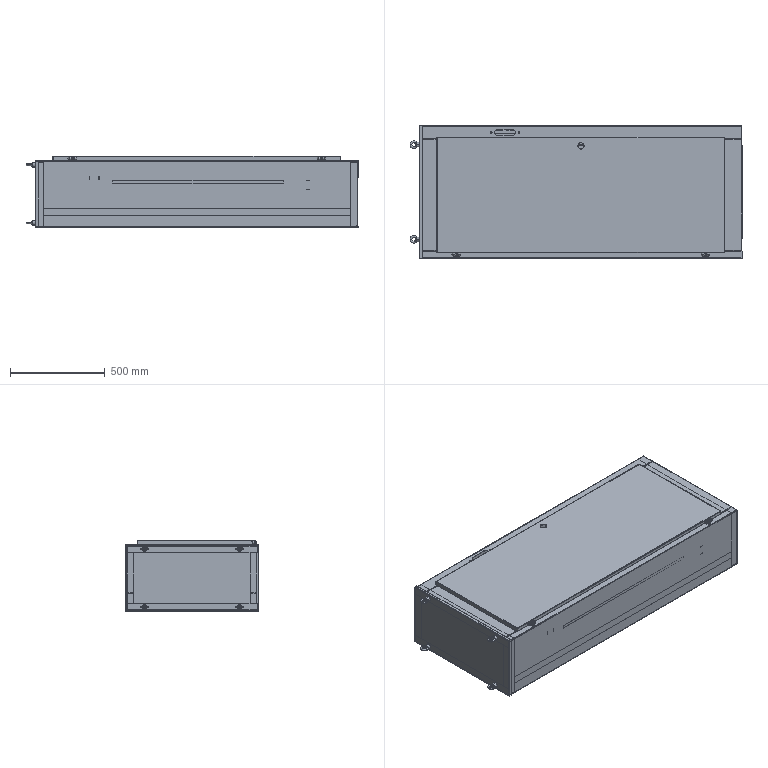Assembly | SolidWorks | mm | 36 component files | 36 solids | 1357 faces | box 1751.5 x 706 x 376.5 mm | volume 10810563 mm3 | plane 653 | cylinder 586 | spline 74 | torus 16 | cone 16 | sphere 12 | commonest cylinder face diameters 8 x154 9 x108 12 x108 7 x46 2 x30 6 x26 5 x25 2.667 x24
Bill of materials:
BeamMountingAngleSteel | 2 |  | Long, slender angle (L-section) with equal-looking legs and a series of evenly spaced, elongated slots along one leg.
CableClamp | 2 |  | U-shaped bent bracket: a flat web with two parallel flanges at right angles, and one round hole through the center of the web.
Door | 1 |  | Thin, flat rectangular plate with one round through-hole near one long edge, roughly midway along it, and small holes in the narrow edge faces.
BeamAngleSteel | 4 |  | Long angle (L-section) with two elongated slots in one leg, one near each end.
LeftAndRightSideAngleSteel | 4 |  | Short angle (L-section) whose two legs differ in length along the part axis: one leg is shorter and set inward from both ends of the other.
FrontUpperAndLowerSill | 2 |  | Elongated sheet-metal cover or tray: a flat top panel with downturned side walls along most of its length, and an unflanged section of the top panel that runs past the walls at one end.
GroundingCopperBlock | 1 |  | Thick, square, flat plate or washer-like block with one central round through-hole.
GroundingDevice | 1 |  | Sheet-metal U-channel clip: a flat web with two parallel flanges, one round hole in the web, and chamfered corners on the flange tips.
Hinge1 | 4 |  | Turned stud or knob: a cylindrical body with a hemispherical dome at one end, and a smaller-diameter externally threaded shank with a short plain neck at the other end.
Hinge2 | 2 |  | Eye-type threaded stud: a domed cylindrical head with flat parallel side faces and a cross hole through it, on a coaxial externally threaded shank.
Pin | 2 |  | Plain solid cylindrical pin or rod with small chamfers or edge breaks at both ends.
LeftSidePlate | 1 |  | Long sheet-metal lipped channel: a tall web with top and bottom return flanges of unequal width, each ending in a short lip, plus small holes along the top flange.
M12LiftingEye | 4 |  | Eye-bolt-like part: a round toroidal ring joined to a tapered cylindrical collar, with a smaller-diameter externally grooved (thread-like) stud extending coaxially from the flat end face of the collar.
RearBackPlate | 1 |  | Long, thin rectangular sheet with short flanges bent down along both long edges, forming a shallow open channel or tray.
RightSidePlate | 1 |  | Long thin-wall lipped C-channel: a tall web with two flanges on the same side, each ending in a short inward-turned return lip. One flange has an elongated slot with two small holes beside it.
SideFixedMountingAngleSteel | 2 |  | Long thin L-shaped (angle) profile with a radiused inside bend. One leg has a single row of evenly spaced elongated slots running along its length.
TerminalPlate | 1 |  | Long narrow bent strip with one obtuse-angle bend, giving a short straight leg and a longer angled leg. A row of evenly spaced elongated slots runs along the length.
TopCoverPlate | 1 |  | Flat rectangular plate with four small round through-holes, one near each corner in a rectangular pattern.
Mates:
1. coincident | RearBackPlate-1 face at (-927.848, -105.605, 13) dir (0, -1, 0) | LeftSidePlate-1 face at (-927.848, -105.605, 0) dir (0, 1, 0)
2. coincident | RearBackPlate-1 face at (-927.848, 394.395, -2) dir (-1, 0, 0) | LeftSidePlate-1 face at (-927.848, -105.605, -2) dir (-1, 0, 0)
3. coincident | RearBackPlate-1 face at (772.152, -105.605, -2) dir (0, 0, -1) | LeftSidePlate-1 face at (-927.848, -203.605, -2) dir (0, 0, -1)
4. coincident | RearBackPlate-1 face at (772.152, 394.395, 13) dir (0, 1, 0) | RightSidePlate-1 face at (772.152, 394.395, 0) dir (0, -1, 0)
5. coincident | RearBackPlate-1 face at (-927.848, 394.395, -2) dir (-1, 0, 0) | RightSidePlate-1 face at (-927.848, 492.395, -2) dir (-1, 0, 0)
6. coincident | RearBackPlate-1 face at (772.152, -105.605, -2) dir (0, 0, -1) | RightSidePlate-1 face at (-927.848, 394.395, -2) dir (0, 0, -1)
7. coincident | LeftSidePlate-1 face at (772.152, -165.605, 346) dir (0, 1, 0) | FrontUpperAndLowerSill-1 face at (-827.848, -165.605, 323) dir (0, -1, 0)
8. coincident | LeftSidePlate-1 face at (772.152, -203.605, 348) dir (0, 0, 1) | FrontUpperAndLowerSill-1 face at (-927.848, -165.605, 348) dir (0, 0, 1)
9. coincident | LeftSidePlate-1 face at (-927.848, -203.605, 348) dir (-1, 0, 0) | FrontUpperAndLowerSill-1 face at (-927.848, 424.395, 346) dir (-1, 0, 0)
10. coincident | RightSidePlate-1 face at (-927.848, 424.395, 346) dir (0, -1, 0) | FrontUpperAndLowerSill-2 face at (672.152, 424.395, 323) dir (0, 1, 0)
11. coincident | RightSidePlate-1 face at (772.152, 424.395, 348) dir (0, 0, 1) | FrontUpperAndLowerSill-2 face at (772.152, 424.395, 348) dir (0, 0, 1)
12. coincident | RightSidePlate-1 face at (772.152, 492.395, 348) dir (1, 0, 0) | FrontUpperAndLowerSill-2 face at (772.152, -165.605, 346) dir (1, 0, 0)
13. coincident | FrontUpperAndLowerSill-1 face at (-927.848, -165.605, 346) dir (0, 0, -1) | FrameAssembly-1/BeamAngleSteel-2 face at (-927.848, 492.395, 346) dir (0, 0, 1)
14. coincident | RightSidePlate-1 face at (-927.848, 492.395, 348) dir (0, -1, 0) | FrameAssembly-1/LeftAndRightSideAngleSteel-1 face at (-887.848, 492.395, 342) dir (0, 1, 0)
15. coincident | FrontUpperAndLowerSill-1 face at (-927.848, 424.395, 346) dir (-1, 0, 0) | FrameAssembly-1/BeamAngleSteel-2 face at (-927.848, 492.395, 306) dir (-1, 0, 0)
16. coincident | RearBackPlate-1 face at (772.152, -105.605, 0) dir (0, 0, 1) | FrameAssembly-2/BeamAngleSteel-1 face at (772.152, 492.395, 0) dir (0, 0, -1)
17. coincident | FrontUpperAndLowerSill-2 face at (772.152, -165.605, 346) dir (1, 0, 0) | FrameAssembly-2/BeamAngleSteel-2 face at (772.152, -203.605, 306) dir (1, 0, 0)
18. coincident | LeftSidePlate-1 face at (772.152, -203.605, -2) dir (0, 1, 0) | FrameAssembly-2/LeftAndRightSideAngleSteel-1 face at (732.152, -203.605, 342) dir (0, -1, 0)
19. distance | TopCoverPlate-1 face at (-914.348, -208.105, -3) dir (0, 0, 1) | RearBackPlate-1 face at (772.152, -105.605, -2) dir (0, 0, -1)
20. distance | TopCoverPlate-1 face at (-914.348, -206.605, 351.5) dir (0, 1, 0) | LeftSidePlate-1 face at (772.152, -205.605, -2) dir (0, -1, 0)
21. coincident | FrameAssembly-1/BeamAngleSteel-2 face at (-927.848, 492.395, 306) dir (-1, 0, 0) | TopCoverPlate-1 face at (-927.848, 497.895, -4.5) dir (1, 0, 0)
22. concentric | TopCoverPlate-1 face at (-927.848, -105.105, 20.5) dir (1, 0, 0) r 6 | M12LiftingEye-1 face at (-904.348, -105.105, 20.5) dir (-1, 0, 0) r 6
23. coincident | TopCoverPlate-1 face at (-929.348, 497.895, -4.5) dir (-1, 0, 0) | M12LiftingEye-1 face at (-929.348, -105.105, 20.5) dir (1, 0, 0)
24. concentric | TopCoverPlate-1 face at (-927.848, -105.105, 326.5) dir (1, 0, 0) r 6 | M12LiftingEye-2 face at (-904.348, -105.105, 326.5) dir (-1, 0, 0) r 6
25. coincident | TopCoverPlate-1 face at (-929.348, 497.895, -4.5) dir (-1, 0, 0) | M12LiftingEye-2 face at (-929.348, -105.105, 326.5) dir (1, 0, 0)
26. concentric | TopCoverPlate-1 face at (-927.848, 394.895, 20.5) dir (1, 0, 0) r 6 | M12LiftingEye-3 face at (-904.348, 394.895, 20.5) dir (-1, 0, 0) r 6
27. coincident | TopCoverPlate-1 face at (-929.348, 497.895, -4.5) dir (-1, 0, 0) | M12LiftingEye-3 face at (-929.348, 394.895, 20.5) dir (1, 0, 0)
28. concentric | TopCoverPlate-1 face at (-927.848, 394.895, 326.5) dir (1, 0, 0) r 6 | M12LiftingEye-4 face at (-904.348, 394.895, 326.5) dir (-1, 0, 0) r 6
29. coincident | TopCoverPlate-1 face at (-929.348, 497.895, -4.5) dir (-1, 0, 0) | M12LiftingEye-4 face at (-929.348, 394.895, 326.5) dir (1, 0, 0)
30. distance | Door-1 face at (682.152, 434.395, 352) dir (1, 0, 0) | FrontUpperAndLowerSill-2 face at (772.152, -165.605, 346) dir (1, 0, 0)
31. distance | LeftSidePlate-1 face at (772.152, -205.605, -2) dir (0, -1, 0) | Door-1 face at (682.152, -175.605, 352) dir (0, -1, 0)
32. concentric | Door-1 face at (-748.848, -173.605, 361) dir (0, -1, 0) r 4.25 | HingeAssembly-1/Hinge1-2 face at (-748.848, -160.605, 361) dir (0, -1, 0) r 4
33. coincident | Door-1 face at (682.152, -175.605, 352) dir (0, -1, 0) | HingeAssembly-1/Hinge1-2 face at (-748.848, -175.605, 361) dir (0, 1, 0)
34. distance | Door-1 face at (682.152, 2858.303, 352) dir (0, 0, -1) | LeftSidePlate-1 face at (772.152, -203.605, 348) dir (0, 0, 1)
35. concentric | Door-1 face at (565.152, -173.605, 361) dir (0, -1, 0) r 4.25 | HingeAssembly-3/Hinge1-2 face at (565.152, -160.605, 361) dir (0, -1, 0) r 4
36. coincident | Door-1 face at (682.152, -175.605, 352) dir (0, -1, 0) | HingeAssembly-3/Hinge1-2 face at (565.152, -175.605, 361) dir (0, 1, 0)
37. coincident | LeftSidePlate-1 face at (772.152, -203.605, -2) dir (0, 1, 0) | SideFixedMountingAngleSteel-1 face at (768.152, -203.605, 98) dir (0, -1, 0)
38. distance | SideFixedMountingAngleSteel-1 face at (768.152, -163.605, 98) dir (0, 0, 1) | LeftSidePlate-1 face at (-927.848, -203.605, 0) dir (0, 0, 1)
39. coincident | FrameAssembly-2/LeftAndRightSideAngleSteel-1 face at (768.152, -196.105, 342) dir (-1, 0, 0) | SideFixedMountingAngleSteel-1 face at (768.152, -164.938, 95.333) dir (1, 0, 0)
40. coincident | RightSidePlate-1 face at (-927.848, 492.395, 348) dir (0, -1, 0) | SideFixedMountingAngleSteel-2 face at (-923.848, 492.395, 98) dir (0, 1, 0)
41. distance | SideFixedMountingAngleSteel-2 face at (-923.848, 452.395, 98) dir (0, 0, 1) | RightSidePlate-1 face at (-927.848, 394.395, 0) dir (0, 0, 1)
42. coincident | FrameAssembly-2/LeftAndRightSideAngleSteel-2 face at (768.152, 484.895, 4) dir (-1, 0, 0) | SideFixedMountingAngleSteel-2 face at (768.152, 453.728, 95.333) dir (1, 0, 0)
43. coincident | SideFixedMountingAngleSteel-1 face at (768.152, -164.938, 94) dir (0, 0, -1) | BeamMountingAngleSteel-1 face at (-644.255, 485.395, 94) dir (0, 0, 1)
44. distance | BeamMountingAngleSteel-1 face at (-642.921, -194.605, 91.333) dir (0, -1, 0) | SideFixedMountingAngleSteel-1 face at (768.152, -199.605, 90.5) dir (0, 1, 0)
45. coincident | SideFixedMountingAngleSteel-1 face at (768.152, -164.938, 94) dir (0, 0, -1) | BeamMountingAngleSteel-2 face at (-325.308, -196.605, 94) dir (0, 0, 1)
46. distance | BeamMountingAngleSteel-2 face at (-326.641, 483.395, 91.333) dir (0, 1, 0) | SideFixedMountingAngleSteel-2 face at (-923.848, 488.395, 90.5) dir (0, -1, 0)
47. coincident | LeftSidePlate-1 face at (772.152, -203.605, -2) dir (0, 1, 0) | TerminalPlate-1 face at (-521.848, -203.605, 231) dir (0, -1, 0)
48. distance | TerminalPlate-1 face at (-521.848, -201.605, 246) dir (0, 0, 1) | LeftSidePlate-1 face at (772.152, -203.605, 346) dir (0, 0, -1)
49. distance | FrameAssembly-2/LeftAndRightSideAngleSteel-1 face at (768.152, -196.105, 342) dir (-1, 0, 0) | TerminalPlate-1 face at (378.152, -179.024, 199.381) dir (1, 0, 0)
50. coincident | FrameAssembly-2/LeftAndRightSideAngleSteel-1 face at (768.152, -196.105, 342) dir (-1, 0, 0) | GroundingDeviceAssembly-1/GroundingDevice-1 face at (768.152, -164.605, 262) dir (1, 0, 0)
51. coincident | FrameAssembly-2/LeftAndRightSideAngleSteel-1 face at (733.486, -199.605, 342) dir (0, 1, 0) | GroundingDeviceAssembly-1/GroundingDevice-1 face at (768.152, -199.605, 262) dir (0, -1, 0)
52. distance | GroundingDeviceAssembly-1/GroundingDevice-1 face at (768.152, -164.605, 262) dir (0, 0, 1) | FrameAssembly-2/BeamAngleSteel-2 face at (764.652, -203.605, 342) dir (0, 0, -1)
53. coincident | LeftSidePlate-1 face at (772.152, -203.605, -2) dir (0, 1, 0) | CableClamp-1 face at (-643.848, -203.605, 266) dir (0, -1, 0)
54. distance | CableClamp-1 face at (-643.848, -190.605, 266) dir (0, 0, 1) | LeftSidePlate-1 face at (772.152, -203.605, 346) dir (0, 0, -1)
55. distance | CableClamp-1 face at (-643.848, -203.605, 266) dir (-1, 0, 0) | FrameAssembly-1/LeftAndRightSideAngleSteel-2 face at (-923.848, -196.105, 4) dir (1, 0, 0)
56. coincident | LeftSidePlate-1 face at (772.152, -203.605, -2) dir (0, 1, 0) | CableClamp-2 face at (515.152, -203.605, 246) dir (0, -1, 0)
57. distance | CableClamp-2 face at (498.152, -203.605, 246) dir (-1, 0, 0) | TerminalPlate-1 face at (378.152, -179.024, 199.381) dir (1, 0, 0)
58. distance | CableClamp-2 face at (515.152, -203.605, 246) dir (0, 0, 1) | LeftSidePlate-1 face at (772.152, -203.605, 346) dir (0, 0, -1)
59. coincident | BeamAngleSteel-1 face at (304.234, 43.454, 18.667) dir (0, 1, 0) | LeftAndRightSideAngleSteel-1 face at (-384.266, 43.454, 322) dir (0, 1, 0)
60. coincident | BeamAngleSteel-1 face at (-391.766, 42.121, 18.667) dir (-1, 0, 0) | LeftAndRightSideAngleSteel-1 face at (-391.766, 79.454, 322) dir (-1, 0, 0)
61. coincident | BeamAngleSteel-1 face at (304.234, 46.954, -16) dir (0, 0, 1) | LeftAndRightSideAngleSteel-1 face at (-389.1, 78.121, -16) dir (0, 0, -1)
62. coincident | BeamAngleSteel-1 face at (304.234, 43.454, 18.667) dir (0, 1, 0) | LeftAndRightSideAngleSteel-2 face at (296.734, 43.454, -16) dir (0, 1, 0)
63. coincident | BeamAngleSteel-1 face at (304.234, 42.121, 18.667) dir (1, 0, 0) | LeftAndRightSideAngleSteel-2 face at (304.234, 79.454, -16) dir (1, 0, 0)
64. coincident | BeamAngleSteel-1 face at (304.234, 46.954, -16) dir (0, 0, 1) | LeftAndRightSideAngleSteel-2 face at (301.567, 78.121, -16) dir (0, 0, -1)
65. coincident | LeftAndRightSideAngleSteel-1 face at (-384.266, 43.454, 322) dir (0, 1, 0) | BeamAngleSteel-2 face at (-391.766, 43.454, 287.333) dir (0, 1, 0)
66. coincident | LeftAndRightSideAngleSteel-1 face at (-391.766, 79.454, 322) dir (-1, 0, 0) | BeamAngleSteel-2 face at (-391.766, 42.121, 287.333) dir (-1, 0, 0)
67. coincident | LeftAndRightSideAngleSteel-1 face at (-389.1, 78.121, 322) dir (0, 0, 1) | BeamAngleSteel-2 face at (-391.766, 46.954, 322) dir (0, 0, -1)
68. coincident | GroundingDevice-1 face at (14.38, -20.277, -2) dir (0, 0, -1) | GroundingCopperBlock-1 face at (-19.687, -16.71, -2) dir (0, 0, 1)
69. concentric | GroundingDevice-1 face at (-5.62, -2.777, 1) dir (0, 0, -1) r 5 | GroundingCopperBlock-1 face at (-5.62, -2.777, -7) dir (0, 0, 1) r 4.25
70. concentric | Hinge2-1 face at (-2.221, -8.361, 9) dir (0, 1, 0) r 4 | Pin-1 face at (-2.221, 14.639, 9) dir (0, -1, 0) r 4
71. distance | Pin-1 face at (-2.221, -15.361, 9) dir (0, -1, 0) | Hinge2-1 face at (60.717, -7.361, 22) dir (0, -1, 0)
72. concentric | Pin-1 face at (-2.221, 14.639, 9) dir (0, -1, 0) r 4 | Hinge1-1 face at (-2.221, 14.639, 9) dir (0, -1, 0) r 4
73. coincident | Hinge2-1 face at (57.987, 6.639, 22) dir (0, 1, 0) | Hinge1-1 face at (-11.221, 6.639, -48.171) dir (0, -1, 0)
74. concentric | Pin-1 face at (-2.221, 14.639, 9) dir (0, -1, 0) r 4 | Hinge1-2 face at (-2.221, -15.361, 9) dir (0, 1, 0) r 4
75. coincident | Hinge2-1 face at (60.717, -7.361, 22) dir (0, -1, 0) | Hinge1-2 face at (-11.221, -7.361, 66.171) dir (0, 1, 0)